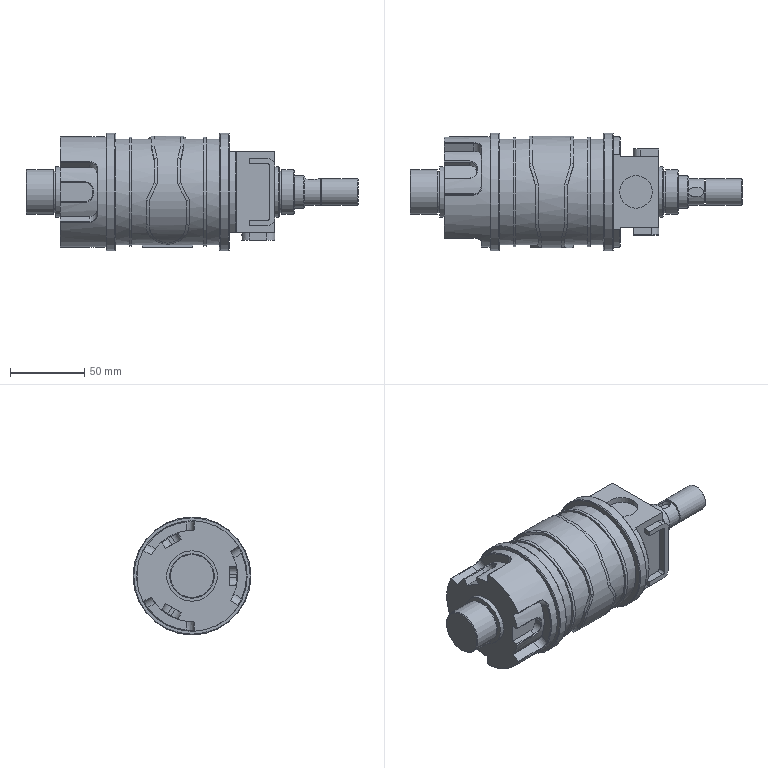Component | NX | DRIVE_SHAFT | 1 solid | 235 faces | volume 597969 mm3 | plane 107 | spline 59 | cylinder 52 | cone 17 | commonest cylinder face diameters 10 x16 3 x4 11 x4 71.5 x3 74.5 x3 61.5 x3 75.5 x2 74 x2